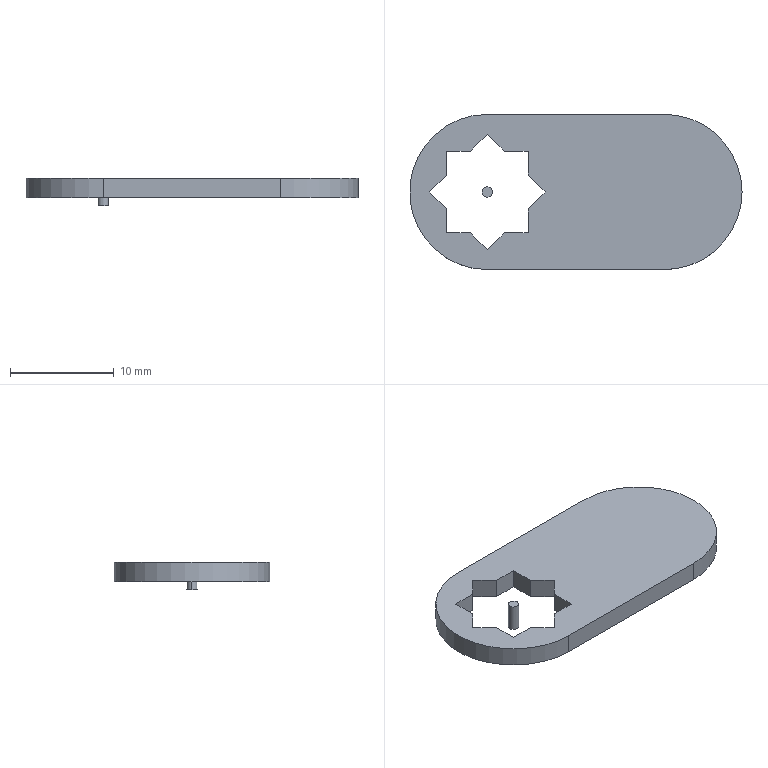Component | SolidWorks | PC-CAJ-P08-1_Lengueta Chapa Guantera Duesco B-1 | 2 solids | 27 faces | box 32 x 14.95 x 2.65 mm | volume 682 mm3 | plane 22 | cylinder 5 | commonest cylinder face diameters 14.95 x3 1 x2 | material Plain Carbon Steel
STEP:
#1=COLOUR_RGB('',0.7922,0.8196,0.9333);
#2=FILL_AREA_STYLE_COLOUR('',#1);
#3=FILL_AREA_STYLE('',(#2));
#4=SURFACE_STYLE_FILL_AREA(#3);
#5=SURFACE_SIDE_STYLE('',(#4));
#6=SURFACE_STYLE_USAGE(.BOTH.,#5);
#7=PRESENTATION_STYLE_ASSIGNMENT((#6));
#8=CARTESIAN_POINT('',(-1.142,-0.9449,8.203));
#9=VERTEX_POINT('',#8);
#10=CARTESIAN_POINT('',(-1.102,-0.9449,8.203));
#11=VERTEX_POINT('',#10);
#12=CARTESIAN_POINT('',(-1.122,-0.9449,8.203));
#13=DIRECTION('',(0.,-0.,1.));
#14=DIRECTION('',(-1.,0.,0.));
#15=AXIS2_PLACEMENT_3D('',#12,#13,#14);
#16=CIRCLE('',#15,0.01969);
#17=EDGE_CURVE('',#9,#11,#16,.T.);
#18=ORIENTED_EDGE('',*,*,#17,.T.);
#19=CARTESIAN_POINT('',(-1.102,-0.9449,8.307));
#20=VERTEX_POINT('',#19);
#21=CARTESIAN_POINT('',(-1.102,-0.9449,8.203));
#22=DIRECTION('',(0.,-0.,1.));
#23=VECTOR('',#22,39.37);
#24=LINE('',#21,#23);
#25=EDGE_CURVE('',#11,#20,#24,.T.);
#26=ORIENTED_EDGE('',*,*,#25,.T.);
#27=CARTESIAN_POINT('',(-1.142,-0.9449,8.307));
#28=VERTEX_POINT('',#27);
#29=CARTESIAN_POINT('',(-1.122,-0.9449,8.307));
#30=DIRECTION('',(-0.,0.,-1.));
#31=DIRECTION('',(-1.,0.,0.));
#32=AXIS2_PLACEMENT_3D('',#29,#30,#31);
#33=CIRCLE('',#32,0.01969);
#34=EDGE_CURVE('',#20,#28,#33,.T.);
#35=ORIENTED_EDGE('',*,*,#34,.T.);
#36=CARTESIAN_POINT('',(-1.142,-0.9449,8.203));
#37=DIRECTION('',(0.,-0.,1.));
#38=VECTOR('',#37,39.37);
#39=LINE('',#36,#38);
#40=EDGE_CURVE('',#9,#28,#39,.T.);
#41=ORIENTED_EDGE('',*,*,#40,.F.);
#42=EDGE_LOOP('',(#18,#26,#35,#41));
#43=FACE_OUTER_BOUND('',#42,.T.);
#44=CARTESIAN_POINT('',(-1.122,-0.9449,8.203));
#45=DIRECTION('',(0.,-0.,1.));
#46=DIRECTION('',(-1.,0.,0.));
#47=AXIS2_PLACEMENT_3D('',#44,#45,#46);
#48=CYLINDRICAL_SURFACE('',#47,0.01969);
#49=ADVANCED_FACE('',(#43),#48,.T.);
#50=ORIENTED_EDGE('',*,*,#25,.F.);
#51=CARTESIAN_POINT('',(-1.122,-0.9449,8.203));
#52=DIRECTION('',(0.,-0.,1.));
#53=DIRECTION('',(-1.,0.,0.));
#54=AXIS2_PLACEMENT_3D('',#51,#52,#53);
#55=CIRCLE('',#54,0.01969);
#56=EDGE_CURVE('',#11,#9,#55,.T.);
#57=ORIENTED_EDGE('',*,*,#56,.T.);
#58=ORIENTED_EDGE('',*,*,#40,.T.);
#59=CARTESIAN_POINT('',(-1.122,-0.9449,8.307));
#60=DIRECTION('',(-0.,0.,-1.));
#61=DIRECTION('',(-1.,0.,0.));
#62=AXIS2_PLACEMENT_3D('',#59,#60,#61);
#63=CIRCLE('',#62,0.01969);
#64=EDGE_CURVE('',#28,#20,#63,.T.);
#65=ORIENTED_EDGE('',*,*,#64,.T.);
#66=EDGE_LOOP('',(#50,#57,#58,#65));
#67=FACE_OUTER_BOUND('',#66,.T.);
#68=CARTESIAN_POINT('',(-1.122,-0.9449,8.203));
#69=DIRECTION('',(0.,-0.,1.));
#70=DIRECTION('',(-1.,0.,0.));
#71=AXIS2_PLACEMENT_3D('',#68,#69,#70);
#72=CYLINDRICAL_SURFACE('',#71,0.01969);
#73=ADVANCED_FACE('',(#67),#72,.T.);
#74=ORIENTED_EDGE('',*,*,#64,.F.);
#75=ORIENTED_EDGE('',*,*,#34,.F.);
#76=EDGE_LOOP('',(#74,#75));
#77=FACE_OUTER_BOUND('',#76,.T.);
#78=CARTESIAN_POINT('',(-1.102,-0.9248,8.307));
#79=DIRECTION('',(0.,-0.,1.));
#80=DIRECTION('',(-1.,0.,0.));
#81=AXIS2_PLACEMENT_3D('',#78,#79,#80);
#82=PLANE('',#81);
#83=ADVANCED_FACE('',(#77),#82,.T.);
#84=ORIENTED_EDGE('',*,*,#17,.F.);
#85=ORIENTED_EDGE('',*,*,#56,.F.);
#86=EDGE_LOOP('',(#84,#85));
#87=FACE_OUTER_BOUND('',#86,.T.);
#88=CARTESIAN_POINT('',(-1.142,-0.9248,8.203));
#89=DIRECTION('',(-0.,0.,-1.));
#90=DIRECTION('',(1.,-0.,-0.));
#91=AXIS2_PLACEMENT_3D('',#88,#89,#90);
#92=PLANE('',#91);
#93=ADVANCED_FACE('',(#87),#92,.T.);
#94=CLOSED_SHELL('',(#49,#73,#83,#93));
#95=MANIFOLD_SOLID_BREP('',#94);
#96=STYLED_ITEM('',(#7),#95);
#97=PRESENTATION_LAYER_ASSIGNMENT('','',(#96));
#98=COLOUR_RGB('',0.7922,0.8196,0.9333);
#99=FILL_AREA_STYLE_COLOUR('',#98);
#100=FILL_AREA_STYLE('',(#99));
#101=SURFACE_STYLE_FILL_AREA(#100);
#102=SURFACE_SIDE_STYLE('',(#101));
#103=SURFACE_STYLE_USAGE(.BOTH.,#102);
#104=PRESENTATION_STYLE_ASSIGNMENT((#103));
#105=CARTESIAN_POINT('',(-0.1565,-0.9449,8.307));
#106=VERTEX_POINT('',#105);
#107=CARTESIAN_POINT('',(-0.4508,-0.6506,8.307));
#108=VERTEX_POINT('',#107);
#109=CARTESIAN_POINT('',(-0.4508,-0.9449,8.307));
#110=DIRECTION('',(0.,-0.,1.));
#111=DIRECTION('',(1.,0.,0.));
#112=AXIS2_PLACEMENT_3D('',#109,#110,#111);
#113=CIRCLE('',#112,0.2943);
#114=EDGE_CURVE('',#106,#108,#113,.T.);
#115=ORIENTED_EDGE('',*,*,#114,.F.);
#116=CARTESIAN_POINT('',(-0.1565,-0.9449,8.232));
#117=VERTEX_POINT('',#116);
#118=CARTESIAN_POINT('',(-0.1565,-0.9449,8.307));
#119=DIRECTION('',(-0.,0.,-1.));
#120=VECTOR('',#119,39.37);
#121=LINE('',#118,#120);
#122=EDGE_CURVE('',#106,#117,#121,.T.);
#123=ORIENTED_EDGE('',*,*,#122,.T.);
#124=CARTESIAN_POINT('',(-0.4508,-0.6506,8.232));
#125=VERTEX_POINT('',#124);
#126=CARTESIAN_POINT('',(-0.4508,-0.9449,8.232));
#127=DIRECTION('',(-0.,0.,-1.));
#128=DIRECTION('',(1.,0.,0.));
#129=AXIS2_PLACEMENT_3D('',#126,#127,#128);
#130=CIRCLE('',#129,0.2943);
#131=EDGE_CURVE('',#125,#117,#130,.T.);
#132=ORIENTED_EDGE('',*,*,#131,.F.);
#133=CARTESIAN_POINT('',(-0.4508,-0.6506,8.27));
#134=DIRECTION('',(-0.,0.,-1.));
#135=VECTOR('',#134,39.37);
#136=LINE('',#133,#135);
#137=EDGE_CURVE('',#108,#125,#136,.T.);
#138=ORIENTED_EDGE('',*,*,#137,.F.);
#139=EDGE_LOOP('',(#115,#123,#132,#138));
#140=FACE_OUTER_BOUND('',#139,.T.);
#141=CARTESIAN_POINT('',(-0.4508,-0.9449,8.307));
#142=DIRECTION('',(-0.,0.,-1.));
#143=DIRECTION('',(1.,0.,0.));
#144=AXIS2_PLACEMENT_3D('',#141,#142,#143);
#145=CYLINDRICAL_SURFACE('',#144,0.2943);
#146=ADVANCED_FACE('',(#140),#145,.T.);
#147=CARTESIAN_POINT('',(-0.9671,-0.79,8.232));
#148=VERTEX_POINT('',#147);
#149=CARTESIAN_POINT('',(-0.9671,-0.79,8.307));
#150=VERTEX_POINT('',#149);
#151=CARTESIAN_POINT('',(-0.9671,-0.79,8.27));
#152=DIRECTION('',(0.,-0.,1.));
#153=VECTOR('',#152,39.37);
#154=LINE('',#151,#153);
#155=EDGE_CURVE('',#148,#150,#154,.T.);
#156=ORIENTED_EDGE('',*,*,#155,.T.);
#157=CARTESIAN_POINT('',(-1.058,-0.79,8.307));
#158=VERTEX_POINT('',#157);
#159=CARTESIAN_POINT('',(-1.013,-0.79,8.307));
#160=DIRECTION('',(-1.,0.,0.));
#161=VECTOR('',#160,39.37);
#162=LINE('',#159,#161);
#163=EDGE_CURVE('',#150,#158,#162,.T.);
#164=ORIENTED_EDGE('',*,*,#163,.T.);
#165=CARTESIAN_POINT('',(-1.058,-0.79,8.232));
#166=VERTEX_POINT('',#165);
#167=CARTESIAN_POINT('',(-1.058,-0.79,8.27));
#168=DIRECTION('',(-0.,0.,-1.));
#169=VECTOR('',#168,39.37);
#170=LINE('',#167,#169);
#171=EDGE_CURVE('',#158,#166,#170,.T.);
#172=ORIENTED_EDGE('',*,*,#171,.T.);
#173=CARTESIAN_POINT('',(-1.013,-0.79,8.232));
#174=DIRECTION('',(1.,-0.,-0.));
#175=VECTOR('',#174,39.37);
#176=LINE('',#173,#175);
#177=EDGE_CURVE('',#166,#148,#176,.T.);
#178=ORIENTED_EDGE('',*,*,#177,.T.);
#179=EDGE_LOOP('',(#156,#164,#172,#178));
#180=FACE_OUTER_BOUND('',#179,.T.);
#181=CARTESIAN_POINT('',(-0.9671,-0.79,8.307));
#182=DIRECTION('',(-0.,-1.,-0.));
#183=DIRECTION('',(-1.,0.,0.));
#184=AXIS2_PLACEMENT_3D('',#181,#182,#183);
#185=PLANE('',#184);
#186=ADVANCED_FACE('',(#180),#185,.T.);
#187=CARTESIAN_POINT('',(-0.9671,-0.8807,8.307));
#188=VERTEX_POINT('',#187);
#189=CARTESIAN_POINT('',(-0.903,-0.9449,8.307));
#190=VERTEX_POINT('',#189);
#191=CARTESIAN_POINT('',(-0.9671,-0.8807,8.307));
#192=DIRECTION('',(0.7071,-0.7071,-0.));
#193=VECTOR('',#192,39.37);
#194=LINE('',#191,#193);
#195=EDGE_CURVE('',#188,#190,#194,.T.);
#196=ORIENTED_EDGE('',*,*,#195,.T.);
#197=CARTESIAN_POINT('',(-0.9671,-1.009,8.307));
#198=VERTEX_POINT('',#197);
#199=CARTESIAN_POINT('',(-0.903,-0.9449,8.307));
#200=DIRECTION('',(-0.7071,-0.7071,-0.));
#201=VECTOR('',#200,39.37);
#202=LINE('',#199,#201);
#203=EDGE_CURVE('',#190,#198,#202,.T.);
#204=ORIENTED_EDGE('',*,*,#203,.T.);
#205=CARTESIAN_POINT('',(-0.9671,-1.1,8.307));
#206=VERTEX_POINT('',#205);
#207=CARTESIAN_POINT('',(-0.9671,-0.9449,8.307));
#208=DIRECTION('',(-0.,-1.,-0.));
#209=VECTOR('',#208,39.37);
#210=LINE('',#207,#209);
#211=EDGE_CURVE('',#198,#206,#210,.T.);
#212=ORIENTED_EDGE('',*,*,#211,.T.);
#213=CARTESIAN_POINT('',(-1.058,-1.1,8.307));
#214=VERTEX_POINT('',#213);
#215=CARTESIAN_POINT('',(-0.7864,-1.1,8.307));
#216=DIRECTION('',(-1.,0.,0.));
#217=VECTOR('',#216,39.37);
#218=LINE('',#215,#217);
#219=EDGE_CURVE('',#206,#214,#218,.T.);
#220=ORIENTED_EDGE('',*,*,#219,.T.);
#221=CARTESIAN_POINT('',(-1.122,-1.164,8.307));
#222=VERTEX_POINT('',#221);
#223=CARTESIAN_POINT('',(-1.058,-1.1,8.307));
#224=DIRECTION('',(-0.7071,-0.7071,-0.));
#225=VECTOR('',#224,39.37);
#226=LINE('',#223,#225);
#227=EDGE_CURVE('',#214,#222,#226,.T.);
#228=ORIENTED_EDGE('',*,*,#227,.T.);
#229=CARTESIAN_POINT('',(-1.186,-1.1,8.307));
#230=VERTEX_POINT('',#229);
#231=CARTESIAN_POINT('',(-1.122,-1.164,8.307));
#232=DIRECTION('',(-0.7071,0.7071,0.));
#233=VECTOR('',#232,39.37);
#234=LINE('',#231,#233);
#235=EDGE_CURVE('',#222,#230,#234,.T.);
#236=ORIENTED_EDGE('',*,*,#235,.T.);
#237=CARTESIAN_POINT('',(-1.277,-1.1,8.307));
#238=VERTEX_POINT('',#237);
#239=CARTESIAN_POINT('',(-0.7864,-1.1,8.307));
#240=DIRECTION('',(-1.,0.,0.));
#241=VECTOR('',#240,39.37);
#242=LINE('',#239,#241);
#243=EDGE_CURVE('',#230,#238,#242,.T.);
#244=ORIENTED_EDGE('',*,*,#243,.T.);
#245=CARTESIAN_POINT('',(-1.277,-1.009,8.307));
#246=VERTEX_POINT('',#245);
#247=CARTESIAN_POINT('',(-1.277,-0.9449,8.307));
#248=DIRECTION('',(0.,1.,0.));
#249=VECTOR('',#248,39.37);
#250=LINE('',#247,#249);
#251=EDGE_CURVE('',#238,#246,#250,.T.);
#252=ORIENTED_EDGE('',*,*,#251,.T.);
#253=CARTESIAN_POINT('',(-1.341,-0.9449,8.307));
#254=VERTEX_POINT('',#253);
#255=CARTESIAN_POINT('',(-1.277,-1.009,8.307));
#256=DIRECTION('',(-0.7071,0.7071,0.));
#257=VECTOR('',#256,39.37);
#258=LINE('',#255,#257);
#259=EDGE_CURVE('',#246,#254,#258,.T.);
#260=ORIENTED_EDGE('',*,*,#259,.T.);
#261=CARTESIAN_POINT('',(-1.277,-0.8807,8.307));
#262=VERTEX_POINT('',#261);
#263=CARTESIAN_POINT('',(-1.341,-0.9449,8.307));
#264=DIRECTION('',(0.7071,0.7071,0.));
#265=VECTOR('',#264,39.37);
#266=LINE('',#263,#265);
#267=EDGE_CURVE('',#254,#262,#266,.T.);
#268=ORIENTED_EDGE('',*,*,#267,.T.);
#269=CARTESIAN_POINT('',(-1.277,-0.79,8.307));
#270=VERTEX_POINT('',#269);
#271=CARTESIAN_POINT('',(-1.277,-0.9449,8.307));
#272=DIRECTION('',(0.,1.,0.));
#273=VECTOR('',#272,39.37);
#274=LINE('',#271,#273);
#275=EDGE_CURVE('',#262,#270,#274,.T.);
#276=ORIENTED_EDGE('',*,*,#275,.T.);
#277=CARTESIAN_POINT('',(-1.186,-0.79,8.307));
#278=VERTEX_POINT('',#277);
#279=CARTESIAN_POINT('',(-0.7864,-0.79,8.307));
#280=DIRECTION('',(1.,-0.,-0.));
#281=VECTOR('',#280,39.37);
#282=LINE('',#279,#281);
#283=EDGE_CURVE('',#270,#278,#282,.T.);
#284=ORIENTED_EDGE('',*,*,#283,.T.);
#285=CARTESIAN_POINT('',(-1.122,-0.7258,8.307));
#286=VERTEX_POINT('',#285);
#287=CARTESIAN_POINT('',(-1.186,-0.79,8.307));
#288=DIRECTION('',(0.7071,0.7071,0.));
#289=VECTOR('',#288,39.37);
#290=LINE('',#287,#289);
#291=EDGE_CURVE('',#278,#286,#290,.T.);
#292=ORIENTED_EDGE('',*,*,#291,.T.);
#293=CARTESIAN_POINT('',(-1.122,-0.7258,8.307));
#294=DIRECTION('',(0.7071,-0.7071,-0.));
#295=VECTOR('',#294,39.37);
#296=LINE('',#293,#295);
#297=EDGE_CURVE('',#286,#158,#296,.T.);
#298=ORIENTED_EDGE('',*,*,#297,.T.);
#299=ORIENTED_EDGE('',*,*,#163,.F.);
#300=CARTESIAN_POINT('',(-0.9671,-0.9449,8.307));
#301=DIRECTION('',(-0.,-1.,-0.));
#302=VECTOR('',#301,39.37);
#303=LINE('',#300,#302);
#304=EDGE_CURVE('',#150,#188,#303,.T.);
#305=ORIENTED_EDGE('',*,*,#304,.T.);
#306=EDGE_LOOP('',(#196,#204,#212,#220,#228,#236,#244,#252,#260,#268,#276,#284,#292,#298,#299,#305));
#307=FACE_BOUND('',#306,.T.);
#308=CARTESIAN_POINT('',(-1.122,-0.6506,8.307));
#309=VERTEX_POINT('',#308);
#310=CARTESIAN_POINT('',(-1.122,-1.239,8.307));
#311=VERTEX_POINT('',#310);
#312=CARTESIAN_POINT('',(-1.122,-0.9449,8.307));
#313=DIRECTION('',(0.,-0.,1.));
#314=DIRECTION('',(1.,0.,0.));
#315=AXIS2_PLACEMENT_3D('',#312,#313,#314);
#316=CIRCLE('',#315,0.2943);
#317=EDGE_CURVE('',#309,#311,#316,.T.);
#318=ORIENTED_EDGE('',*,*,#317,.T.);
#319=CARTESIAN_POINT('',(-0.4508,-1.239,8.307));
#320=VERTEX_POINT('',#319);
#321=CARTESIAN_POINT('',(-0.7864,-1.239,8.307));
#322=DIRECTION('',(1.,-0.,-0.));
#323=VECTOR('',#322,39.37);
#324=LINE('',#321,#323);
#325=EDGE_CURVE('',#311,#320,#324,.T.);
#326=ORIENTED_EDGE('',*,*,#325,.T.);
#327=CARTESIAN_POINT('',(-0.4508,-0.9449,8.307));
#328=DIRECTION('',(0.,-0.,1.));
#329=DIRECTION('',(1.,0.,0.));
#330=AXIS2_PLACEMENT_3D('',#327,#328,#329);
#331=CIRCLE('',#330,0.2943);
#332=EDGE_CURVE('',#320,#106,#331,.T.);
#333=ORIENTED_EDGE('',*,*,#332,.T.);
#334=ORIENTED_EDGE('',*,*,#114,.T.);
#335=CARTESIAN_POINT('',(-0.7864,-0.6506,8.307));
#336=DIRECTION('',(-1.,0.,0.));
#337=VECTOR('',#336,39.37);
#338=LINE('',#335,#337);
#339=EDGE_CURVE('',#108,#309,#338,.T.);
#340=ORIENTED_EDGE('',*,*,#339,.T.);
#341=EDGE_LOOP('',(#318,#326,#333,#334,#340));
#342=FACE_OUTER_BOUND('',#341,.T.);
#343=CARTESIAN_POINT('',(-0.1439,-0.6506,8.307));
#344=DIRECTION('',(0.,-0.,1.));
#345=DIRECTION('',(-1.,0.,0.));
#346=AXIS2_PLACEMENT_3D('',#343,#344,#345);
#347=PLANE('',#346);
#348=ADVANCED_FACE('',(#307,#342),#347,.T.);
#349=ORIENTED_EDGE('',*,*,#155,.F.);
#350=CARTESIAN_POINT('',(-0.9671,-0.8807,8.232));
#351=VERTEX_POINT('',#350);
#352=CARTESIAN_POINT('',(-0.9671,-0.8353,8.232));
#353=DIRECTION('',(-0.,-1.,-0.));
#354=VECTOR('',#353,39.37);
#355=LINE('',#352,#354);
#356=EDGE_CURVE('',#148,#351,#355,.T.);
#357=ORIENTED_EDGE('',*,*,#356,.T.);
#358=CARTESIAN_POINT('',(-0.9671,-0.8807,8.27));
#359=DIRECTION('',(0.,-0.,1.));
#360=VECTOR('',#359,39.37);
#361=LINE('',#358,#360);
#362=EDGE_CURVE('',#351,#188,#361,.T.);
#363=ORIENTED_EDGE('',*,*,#362,.T.);
#364=ORIENTED_EDGE('',*,*,#304,.F.);
#365=EDGE_LOOP('',(#349,#357,#363,#364));
#366=FACE_OUTER_BOUND('',#365,.T.);
#367=CARTESIAN_POINT('',(-0.9671,-0.8807,8.307));
#368=DIRECTION('',(-1.,0.,0.));
#369=DIRECTION('',(0.,1.,0.));
#370=AXIS2_PLACEMENT_3D('',#367,#368,#369);
#371=PLANE('',#370);
#372=ADVANCED_FACE('',(#366),#371,.T.);
#373=CARTESIAN_POINT('',(-1.122,-1.164,8.232));
#374=VERTEX_POINT('',#373);
#375=CARTESIAN_POINT('',(-1.058,-1.1,8.232));
#376=VERTEX_POINT('',#375);
#377=CARTESIAN_POINT('',(-1.122,-1.164,8.232));
#378=DIRECTION('',(0.7071,0.7071,0.));
#379=VECTOR('',#378,39.37);
#380=LINE('',#377,#379);
#381=EDGE_CURVE('',#374,#376,#380,.T.);
#382=ORIENTED_EDGE('',*,*,#381,.T.);
#383=CARTESIAN_POINT('',(-0.9671,-1.1,8.232));
#384=VERTEX_POINT('',#383);
#385=CARTESIAN_POINT('',(-0.7864,-1.1,8.232));
#386=DIRECTION('',(1.,-0.,-0.));
#387=VECTOR('',#386,39.37);
#388=LINE('',#385,#387);
#389=EDGE_CURVE('',#376,#384,#388,.T.);
#390=ORIENTED_EDGE('',*,*,#389,.T.);
#391=CARTESIAN_POINT('',(-0.9671,-1.009,8.232));
#392=VERTEX_POINT('',#391);
#393=CARTESIAN_POINT('',(-0.9671,-0.9449,8.232));
#394=DIRECTION('',(0.,1.,0.));
#395=VECTOR('',#394,39.37);
#396=LINE('',#393,#395);
#397=EDGE_CURVE('',#384,#392,#396,.T.);
#398=ORIENTED_EDGE('',*,*,#397,.T.);
#399=CARTESIAN_POINT('',(-0.903,-0.9449,8.232));
#400=VERTEX_POINT('',#399);
#401=CARTESIAN_POINT('',(-0.9671,-1.009,8.232));
#402=DIRECTION('',(0.7071,0.7071,0.));
#403=VECTOR('',#402,39.37);
#404=LINE('',#401,#403);
#405=EDGE_CURVE('',#392,#400,#404,.T.);
#406=ORIENTED_EDGE('',*,*,#405,.T.);
#407=CARTESIAN_POINT('',(-0.903,-0.9449,8.232));
#408=DIRECTION('',(-0.7071,0.7071,0.));
#409=VECTOR('',#408,39.37);
#410=LINE('',#407,#409);
#411=EDGE_CURVE('',#400,#351,#410,.T.);
#412=ORIENTED_EDGE('',*,*,#411,.T.);
#413=ORIENTED_EDGE('',*,*,#356,.F.);
#414=ORIENTED_EDGE('',*,*,#177,.F.);
#415=CARTESIAN_POINT('',(-1.122,-0.7258,8.232));
#416=VERTEX_POINT('',#415);
#417=CARTESIAN_POINT('',(-1.058,-0.79,8.232));
#418=DIRECTION('',(-0.7071,0.7071,0.));
#419=VECTOR('',#418,39.37);
#420=LINE('',#417,#419);
#421=EDGE_CURVE('',#166,#416,#420,.T.);
#422=ORIENTED_EDGE('',*,*,#421,.T.);
#423=CARTESIAN_POINT('',(-1.186,-0.79,8.232));
#424=VERTEX_POINT('',#423);
#425=CARTESIAN_POINT('',(-1.122,-0.7258,8.232));
#426=DIRECTION('',(-0.7071,-0.7071,-0.));
#427=VECTOR('',#426,39.37);
#428=LINE('',#425,#427);
#429=EDGE_CURVE('',#416,#424,#428,.T.);
#430=ORIENTED_EDGE('',*,*,#429,.T.);
#431=CARTESIAN_POINT('',(-1.277,-0.79,8.232));
#432=VERTEX_POINT('',#431);
#433=CARTESIAN_POINT('',(-0.7864,-0.79,8.232));
#434=DIRECTION('',(-1.,0.,0.));
#435=VECTOR('',#434,39.37);
#436=LINE('',#433,#435);
#437=EDGE_CURVE('',#424,#432,#436,.T.);
#438=ORIENTED_EDGE('',*,*,#437,.T.);
#439=CARTESIAN_POINT('',(-1.277,-0.8807,8.232));
#440=VERTEX_POINT('',#439);
#441=CARTESIAN_POINT('',(-1.277,-0.9449,8.232));
#442=DIRECTION('',(-0.,-1.,-0.));
#443=VECTOR('',#442,39.37);
#444=LINE('',#441,#443);
#445=EDGE_CURVE('',#432,#440,#444,.T.);
#446=ORIENTED_EDGE('',*,*,#445,.T.);
#447=CARTESIAN_POINT('',(-1.341,-0.9449,8.232));
#448=VERTEX_POINT('',#447);
#449=CARTESIAN_POINT('',(-1.277,-0.8807,8.232));
#450=DIRECTION('',(-0.7071,-0.7071,-0.));
#451=VECTOR('',#450,39.37);
#452=LINE('',#449,#451);
#453=EDGE_CURVE('',#440,#448,#452,.T.);
#454=ORIENTED_EDGE('',*,*,#453,.T.);
#455=CARTESIAN_POINT('',(-1.277,-1.009,8.232));
#456=VERTEX_POINT('',#455);
#457=CARTESIAN_POINT('',(-1.341,-0.9449,8.232));
#458=DIRECTION('',(0.7071,-0.7071,-0.));
#459=VECTOR('',#458,39.37);
#460=LINE('',#457,#459);
#461=EDGE_CURVE('',#448,#456,#460,.T.);
#462=ORIENTED_EDGE('',*,*,#461,.T.);
#463=CARTESIAN_POINT('',(-1.277,-1.1,8.232));
#464=VERTEX_POINT('',#463);
#465=CARTESIAN_POINT('',(-1.277,-0.9449,8.232));
#466=DIRECTION('',(-0.,-1.,-0.));
#467=VECTOR('',#466,39.37);
#468=LINE('',#465,#467);
#469=EDGE_CURVE('',#456,#464,#468,.T.);
#470=ORIENTED_EDGE('',*,*,#469,.T.);
#471=CARTESIAN_POINT('',(-1.186,-1.1,8.232));
#472=VERTEX_POINT('',#471);
#473=CARTESIAN_POINT('',(-0.7864,-1.1,8.232));
#474=DIRECTION('',(1.,-0.,-0.));
#475=VECTOR('',#474,39.37);
#476=LINE('',#473,#475);
#477=EDGE_CURVE('',#464,#472,#476,.T.);
#478=ORIENTED_EDGE('',*,*,#477,.T.);
#479=CARTESIAN_POINT('',(-1.186,-1.1,8.232));
#480=DIRECTION('',(0.7071,-0.7071,-0.));
#481=VECTOR('',#480,39.37);
#482=LINE('',#479,#481);
#483=EDGE_CURVE('',#472,#374,#482,.T.);
#484=ORIENTED_EDGE('',*,*,#483,.T.);
#485=EDGE_LOOP('',(#382,#390,#398,#406,#412,#413,#414,#422,#430,#438,#446,#454,#462,#470,#478,#484));
#486=FACE_BOUND('',#485,.T.);
#487=CARTESIAN_POINT('',(-1.122,-1.239,8.232));
#488=VERTEX_POINT('',#487);
#489=CARTESIAN_POINT('',(-1.122,-0.6506,8.232));
#490=VERTEX_POINT('',#489);
#491=CARTESIAN_POINT('',(-1.122,-0.9449,8.232));
#492=DIRECTION('',(-0.,0.,-1.));
#493=DIRECTION('',(1.,0.,0.));
#494=AXIS2_PLACEMENT_3D('',#491,#492,#493);
#495=CIRCLE('',#494,0.2943);
#496=EDGE_CURVE('',#488,#490,#495,.T.);
#497=ORIENTED_EDGE('',*,*,#496,.T.);
#498=CARTESIAN_POINT('',(-0.7864,-0.6506,8.232));
#499=DIRECTION('',(1.,-0.,-0.));
#500=VECTOR('',#499,39.37);
#501=LINE('',#498,#500);
#502=EDGE_CURVE('',#490,#125,#501,.T.);
#503=ORIENTED_EDGE('',*,*,#502,.T.);
#504=ORIENTED_EDGE('',*,*,#131,.T.);
#505=CARTESIAN_POINT('',(-0.4508,-1.239,8.232));
#506=VERTEX_POINT('',#505);
#507=CARTESIAN_POINT('',(-0.4508,-0.9449,8.232));
#508=DIRECTION('',(-0.,0.,-1.));
#509=DIRECTION('',(1.,0.,0.));
#510=AXIS2_PLACEMENT_3D('',#507,#508,#509);
#511=CIRCLE('',#510,0.2943);
#512=EDGE_CURVE('',#117,#506,#511,.T.);
#513=ORIENTED_EDGE('',*,*,#512,.T.);
#514=CARTESIAN_POINT('',(-0.7864,-1.239,8.232));
#515=DIRECTION('',(-1.,0.,0.));
#516=VECTOR('',#515,39.37);
#517=LINE('',#514,#516);
#518=EDGE_CURVE('',#506,#488,#517,.T.);
#519=ORIENTED_EDGE('',*,*,#518,.T.);
#520=EDGE_LOOP('',(#497,#503,#504,#513,#519));
#521=FACE_OUTER_BOUND('',#520,.T.);
#522=CARTESIAN_POINT('',(-1.429,-0.6506,8.232));
#523=DIRECTION('',(-0.,0.,-1.));
#524=DIRECTION('',(1.,-0.,-0.));
#525=AXIS2_PLACEMENT_3D('',#522,#523,#524);
#526=PLANE('',#525);
#527=ADVANCED_FACE('',(#486,#521),#526,.T.);
#528=CARTESIAN_POINT('',(-1.122,-0.7258,8.27));
#529=DIRECTION('',(-0.,0.,-1.));
#530=VECTOR('',#529,39.37);
#531=LINE('',#528,#530);
#532=EDGE_CURVE('',#286,#416,#531,.T.);
#533=ORIENTED_EDGE('',*,*,#532,.T.);
#534=ORIENTED_EDGE('',*,*,#421,.F.);
#535=ORIENTED_EDGE('',*,*,#171,.F.);
#536=ORIENTED_EDGE('',*,*,#297,.F.);
#537=EDGE_LOOP('',(#533,#534,#535,#536));
#538=FACE_OUTER_BOUND('',#537,.T.);
#539=CARTESIAN_POINT('',(-1.058,-0.79,8.307));
#540=DIRECTION('',(-0.7071,-0.7071,-0.));
#541=DIRECTION('',(-0.7071,0.7071,0.));
#542=AXIS2_PLACEMENT_3D('',#539,#540,#541);
#543=PLANE('',#542);
#544=ADVANCED_FACE('',(#538),#543,.T.);
#545=CARTESIAN_POINT('',(-0.903,-0.9449,8.27));
#546=DIRECTION('',(-0.,0.,-1.));
#547=VECTOR('',#546,39.37);
#548=LINE('',#545,#547);
#549=EDGE_CURVE('',#190,#400,#548,.T.);
#550=ORIENTED_EDGE('',*,*,#549,.T.);
#551=ORIENTED_EDGE('',*,*,#405,.F.);
#552=CARTESIAN_POINT('',(-0.9671,-1.009,8.27));
#553=DIRECTION('',(0.,-0.,1.));
#554=VECTOR('',#553,39.37);
#555=LINE('',#552,#554);
#556=EDGE_CURVE('',#392,#198,#555,.T.);
#557=ORIENTED_EDGE('',*,*,#556,.T.);
#558=ORIENTED_EDGE('',*,*,#203,.F.);
#559=EDGE_LOOP('',(#550,#551,#557,#558));
#560=FACE_OUTER_BOUND('',#559,.T.);
#561=CARTESIAN_POINT('',(-0.9671,-1.009,8.307));
#562=DIRECTION('',(-0.7071,0.7071,0.));
#563=DIRECTION('',(0.7071,0.7071,0.));
#564=AXIS2_PLACEMENT_3D('',#561,#562,#563);
#565=PLANE('',#564);
#566=ADVANCED_FACE('',(#560),#565,.T.);
#567=ORIENTED_EDGE('',*,*,#549,.F.);
#568=ORIENTED_EDGE('',*,*,#195,.F.);
#569=ORIENTED_EDGE('',*,*,#362,.F.);
#570=ORIENTED_EDGE('',*,*,#411,.F.);
#571=EDGE_LOOP('',(#567,#568,#569,#570));
#572=FACE_OUTER_BOUND('',#571,.T.);
#573=CARTESIAN_POINT('',(-0.903,-0.9449,8.307));
#574=DIRECTION('',(-0.7071,-0.7071,-0.));
#575=DIRECTION('',(-0.7071,0.7071,0.));
#576=AXIS2_PLACEMENT_3D('',#573,#574,#575);
#577=PLANE('',#576);
#578=ADVANCED_FACE('',(#572),#577,.T.);
#579=ORIENTED_EDGE('',*,*,#532,.F.);
#580=ORIENTED_EDGE('',*,*,#291,.F.);
#581=CARTESIAN_POINT('',(-1.186,-0.79,8.27));
#582=DIRECTION('',(-0.,0.,-1.));
#583=VECTOR('',#582,39.37);
#584=LINE('',#581,#583);
#585=EDGE_CURVE('',#278,#424,#584,.T.);
#586=ORIENTED_EDGE('',*,*,#585,.T.);
#587=ORIENTED_EDGE('',*,*,#429,.F.);
#588=EDGE_LOOP('',(#579,#580,#586,#587));
#589=FACE_OUTER_BOUND('',#588,.T.);
#590=CARTESIAN_POINT('',(-1.122,-0.7258,8.307));
#591=DIRECTION('',(0.7071,-0.7071,-0.));
#592=DIRECTION('',(-0.7071,-0.7071,-0.));
#593=AXIS2_PLACEMENT_3D('',#590,#591,#592);
#594=PLANE('',#593);
#595=ADVANCED_FACE('',(#589),#594,.T.);
#596=CARTESIAN_POINT('',(-1.277,-0.79,8.27));
#597=DIRECTION('',(-0.,0.,-1.));
#598=VECTOR('',#597,39.37);
#599=LINE('',#596,#598);
#600=EDGE_CURVE('',#270,#432,#599,.T.);
#601=ORIENTED_EDGE('',*,*,#600,.T.);
#602=ORIENTED_EDGE('',*,*,#437,.F.);
#603=ORIENTED_EDGE('',*,*,#585,.F.);
#604=ORIENTED_EDGE('',*,*,#283,.F.);
#605=EDGE_LOOP('',(#601,#602,#603,#604));
#606=FACE_OUTER_BOUND('',#605,.T.);
#607=CARTESIAN_POINT('',(-1.186,-0.79,8.307));
#608=DIRECTION('',(-0.,-1.,-0.));
#609=DIRECTION('',(-1.,0.,0.));
#610=AXIS2_PLACEMENT_3D('',#607,#608,#609);
#611=PLANE('',#610);
#612=ADVANCED_FACE('',(#606),#611,.T.);
#613=ORIENTED_EDGE('',*,*,#600,.F.);
#614=ORIENTED_EDGE('',*,*,#275,.F.);
#615=CARTESIAN_POINT('',(-1.277,-0.8807,8.27));
#616=DIRECTION('',(-0.,0.,-1.));
#617=VECTOR('',#616,39.37);
#618=LINE('',#615,#617);
#619=EDGE_CURVE('',#262,#440,#618,.T.);
#620=ORIENTED_EDGE('',*,*,#619,.T.);
#621=ORIENTED_EDGE('',*,*,#445,.F.);
#622=EDGE_LOOP('',(#613,#614,#620,#621));
#623=FACE_OUTER_BOUND('',#622,.T.);
#624=CARTESIAN_POINT('',(-1.277,-0.79,8.307));
#625=DIRECTION('',(1.,-0.,-0.));
#626=DIRECTION('',(-0.,-1.,-0.));
#627=AXIS2_PLACEMENT_3D('',#624,#625,#626);
#628=PLANE('',#627);
#629=ADVANCED_FACE('',(#623),#628,.T.);
#630=CARTESIAN_POINT('',(-1.341,-0.9449,8.27));
#631=DIRECTION('',(-0.,0.,-1.));
#632=VECTOR('',#631,39.37);
#633=LINE('',#630,#632);
#634=EDGE_CURVE('',#254,#448,#633,.T.);
#635=ORIENTED_EDGE('',*,*,#634,.T.);
#636=ORIENTED_EDGE('',*,*,#453,.F.);
#637=ORIENTED_EDGE('',*,*,#619,.F.);
#638=ORIENTED_EDGE('',*,*,#267,.F.);
#639=EDGE_LOOP('',(#635,#636,#637,#638));
#640=FACE_OUTER_BOUND('',#639,.T.);
#641=CARTESIAN_POINT('',(-1.277,-0.8807,8.307));
#642=DIRECTION('',(0.7071,-0.7071,-0.));
#643=DIRECTION('',(-0.7071,-0.7071,-0.));
#644=AXIS2_PLACEMENT_3D('',#641,#642,#643);
#645=PLANE('',#644);
#646=ADVANCED_FACE('',(#640),#645,.T.);
#647=ORIENTED_EDGE('',*,*,#634,.F.);
#648=ORIENTED_EDGE('',*,*,#259,.F.);
#649=CARTESIAN_POINT('',(-1.277,-1.009,8.27));
#650=DIRECTION('',(-0.,0.,-1.));
#651=VECTOR('',#650,39.37);
#652=LINE('',#649,#651);
#653=EDGE_CURVE('',#246,#456,#652,.T.);
#654=ORIENTED_EDGE('',*,*,#653,.T.);
#655=ORIENTED_EDGE('',*,*,#461,.F.);
#656=EDGE_LOOP('',(#647,#648,#654,#655));
#657=FACE_OUTER_BOUND('',#656,.T.);
#658=CARTESIAN_POINT('',(-1.341,-0.9449,8.307));
#659=DIRECTION('',(0.7071,0.7071,0.));
#660=DIRECTION('',(0.7071,-0.7071,-0.));
#661=AXIS2_PLACEMENT_3D('',#658,#659,#660);
#662=PLANE('',#661);
#663=ADVANCED_FACE('',(#657),#662,.T.);
#664=CARTESIAN_POINT('',(-1.277,-1.1,8.27));
#665=DIRECTION('',(-0.,0.,-1.));
#666=VECTOR('',#665,39.37);
#667=LINE('',#664,#666);
#668=EDGE_CURVE('',#238,#464,#667,.T.);
#669=ORIENTED_EDGE('',*,*,#668,.T.);
#670=ORIENTED_EDGE('',*,*,#469,.F.);
#671=ORIENTED_EDGE('',*,*,#653,.F.);
#672=ORIENTED_EDGE('',*,*,#251,.F.);
#673=EDGE_LOOP('',(#669,#670,#671,#672));
#674=FACE_OUTER_BOUND('',#673,.T.);
#675=CARTESIAN_POINT('',(-1.277,-1.009,8.307));
#676=DIRECTION('',(1.,-0.,-0.));
#677=DIRECTION('',(-0.,-1.,-0.));
#678=AXIS2_PLACEMENT_3D('',#675,#676,#677);
#679=PLANE('',#678);
#680=ADVANCED_FACE('',(#674),#679,.T.);
#681=ORIENTED_EDGE('',*,*,#668,.F.);
#682=ORIENTED_EDGE('',*,*,#243,.F.);
#683=CARTESIAN_POINT('',(-1.186,-1.1,8.27));
#684=DIRECTION('',(-0.,0.,-1.));
#685=VECTOR('',#684,39.37);
#686=LINE('',#683,#685);
#687=EDGE_CURVE('',#230,#472,#686,.T.);
#688=ORIENTED_EDGE('',*,*,#687,.T.);
#689=ORIENTED_EDGE('',*,*,#477,.F.);
#690=EDGE_LOOP('',(#681,#682,#688,#689));
#691=FACE_OUTER_BOUND('',#690,.T.);
#692=CARTESIAN_POINT('',(-1.277,-1.1,8.307));
#693=DIRECTION('',(0.,1.,0.));
#694=DIRECTION('',(1.,-0.,-0.));
#695=AXIS2_PLACEMENT_3D('',#692,#693,#694);
#696=PLANE('',#695);
#697=ADVANCED_FACE('',(#691),#696,.T.);
#698=CARTESIAN_POINT('',(-1.122,-1.164,8.27));
#699=DIRECTION('',(-0.,0.,-1.));
#700=VECTOR('',#699,39.37);
#701=LINE('',#698,#700);
#702=EDGE_CURVE('',#222,#374,#701,.T.);
#703=ORIENTED_EDGE('',*,*,#702,.T.);
#704=ORIENTED_EDGE('',*,*,#483,.F.);
#705=ORIENTED_EDGE('',*,*,#687,.F.);
#706=ORIENTED_EDGE('',*,*,#235,.F.);
#707=EDGE_LOOP('',(#703,#704,#705,#706));
#708=FACE_OUTER_BOUND('',#707,.T.);
#709=CARTESIAN_POINT('',(-1.186,-1.1,8.307));
#710=DIRECTION('',(0.7071,0.7071,0.));
#711=DIRECTION('',(0.7071,-0.7071,-0.));
#712=AXIS2_PLACEMENT_3D('',#709,#710,#711);
#713=PLANE('',#712);
#714=ADVANCED_FACE('',(#708),#713,.T.);
#715=ORIENTED_EDGE('',*,*,#702,.F.);
#716=ORIENTED_EDGE('',*,*,#227,.F.);
#717=CARTESIAN_POINT('',(-1.058,-1.1,8.27));
#718=DIRECTION('',(-0.,0.,-1.));
#719=VECTOR('',#718,39.37);
#720=LINE('',#717,#719);
#721=EDGE_CURVE('',#214,#376,#720,.T.);
#722=ORIENTED_EDGE('',*,*,#721,.T.);
#723=ORIENTED_EDGE('',*,*,#381,.F.);
#724=EDGE_LOOP('',(#715,#716,#722,#723));
#725=FACE_OUTER_BOUND('',#724,.T.);
#726=CARTESIAN_POINT('',(-1.122,-1.164,8.307));
#727=DIRECTION('',(-0.7071,0.7071,0.));
#728=DIRECTION('',(0.7071,0.7071,0.));
#729=AXIS2_PLACEMENT_3D('',#726,#727,#728);
#730=PLANE('',#729);
#731=ADVANCED_FACE('',(#725),#730,.T.);
#732=CARTESIAN_POINT('',(-0.9671,-1.1,8.27));
#733=DIRECTION('',(-0.,0.,-1.));
#734=VECTOR('',#733,39.37);
#735=LINE('',#732,#734);
#736=EDGE_CURVE('',#206,#384,#735,.T.);
#737=ORIENTED_EDGE('',*,*,#736,.T.);
#738=ORIENTED_EDGE('',*,*,#389,.F.);
#739=ORIENTED_EDGE('',*,*,#721,.F.);
#740=ORIENTED_EDGE('',*,*,#219,.F.);
#741=EDGE_LOOP('',(#737,#738,#739,#740));
#742=FACE_OUTER_BOUND('',#741,.T.);
#743=CARTESIAN_POINT('',(-1.058,-1.1,8.307));
#744=DIRECTION('',(0.,1.,0.));
#745=DIRECTION('',(1.,-0.,-0.));
#746=AXIS2_PLACEMENT_3D('',#743,#744,#745);
#747=PLANE('',#746);
#748=ADVANCED_FACE('',(#742),#747,.T.);
#749=ORIENTED_EDGE('',*,*,#736,.F.);
#750=ORIENTED_EDGE('',*,*,#211,.F.);
#751=ORIENTED_EDGE('',*,*,#556,.F.);
#752=ORIENTED_EDGE('',*,*,#397,.F.);
#753=EDGE_LOOP('',(#749,#750,#751,#752));
#754=FACE_OUTER_BOUND('',#753,.T.);
#755=CARTESIAN_POINT('',(-0.9671,-1.1,8.307));
#756=DIRECTION('',(-1.,0.,0.));
#757=DIRECTION('',(0.,1.,0.));
#758=AXIS2_PLACEMENT_3D('',#755,#756,#757);
#759=PLANE('',#758);
#760=ADVANCED_FACE('',(#754),#759,.T.);
#761=ORIENTED_EDGE('',*,*,#518,.F.);
#762=CARTESIAN_POINT('',(-0.4508,-1.239,8.27));
#763=DIRECTION('',(0.,-0.,1.));
#764=VECTOR('',#763,39.37);
#765=LINE('',#762,#764);
#766=EDGE_CURVE('',#506,#320,#765,.T.);
#767=ORIENTED_EDGE('',*,*,#766,.T.);
#768=ORIENTED_EDGE('',*,*,#325,.F.);
#769=CARTESIAN_POINT('',(-1.122,-1.239,8.27));
#770=DIRECTION('',(-0.,0.,-1.));
#771=VECTOR('',#770,39.37);
#772=LINE('',#769,#771);
#773=EDGE_CURVE('',#311,#488,#772,.T.);
#774=ORIENTED_EDGE('',*,*,#773,.T.);
#775=EDGE_LOOP('',(#761,#767,#768,#774));
#776=FACE_OUTER_BOUND('',#775,.T.);
#777=CARTESIAN_POINT('',(-0.4508,-1.239,8.232));
#778=DIRECTION('',(-0.,-1.,-0.));
#779=DIRECTION('',(0.,-0.,1.));
#780=AXIS2_PLACEMENT_3D('',#777,#778,#779);
#781=PLANE('',#780);
#782=ADVANCED_FACE('',(#776),#781,.T.);
#783=ORIENTED_EDGE('',*,*,#773,.F.);
#784=ORIENTED_EDGE('',*,*,#317,.F.);
#785=CARTESIAN_POINT('',(-1.122,-0.6506,8.27));
#786=DIRECTION('',(-0.,0.,-1.));
#787=VECTOR('',#786,39.37);
#788=LINE('',#785,#787);
#789=EDGE_CURVE('',#309,#490,#788,.T.);
#790=ORIENTED_EDGE('',*,*,#789,.T.);
#791=ORIENTED_EDGE('',*,*,#496,.F.);
#792=EDGE_LOOP('',(#783,#784,#790,#791));
#793=FACE_OUTER_BOUND('',#792,.T.);
#794=CARTESIAN_POINT('',(-1.122,-0.9449,8.307));
#795=DIRECTION('',(-0.,0.,-1.));
#796=DIRECTION('',(1.,0.,0.));
#797=AXIS2_PLACEMENT_3D('',#794,#795,#796);
#798=CYLINDRICAL_SURFACE('',#797,0.2943);
#799=ADVANCED_FACE('',(#793),#798,.T.);
#800=ORIENTED_EDGE('',*,*,#502,.F.);
#801=ORIENTED_EDGE('',*,*,#789,.F.);
#802=ORIENTED_EDGE('',*,*,#339,.F.);
#803=ORIENTED_EDGE('',*,*,#137,.T.);
#804=EDGE_LOOP('',(#800,#801,#802,#803));
#805=FACE_OUTER_BOUND('',#804,.T.);
#806=CARTESIAN_POINT('',(-0.4508,-0.6506,8.307));
#807=DIRECTION('',(0.,1.,0.));
#808=DIRECTION('',(-0.,0.,-1.));
#809=AXIS2_PLACEMENT_3D('',#806,#807,#808);
#810=PLANE('',#809);
#811=ADVANCED_FACE('',(#805),#810,.T.);
#812=ORIENTED_EDGE('',*,*,#122,.F.);
#813=ORIENTED_EDGE('',*,*,#332,.F.);
#814=ORIENTED_EDGE('',*,*,#766,.F.);
#815=ORIENTED_EDGE('',*,*,#512,.F.);
#816=EDGE_LOOP('',(#812,#813,#814,#815));
#817=FACE_OUTER_BOUND('',#816,.T.);
#818=CARTESIAN_POINT('',(-0.4508,-0.9449,8.307));
#819=DIRECTION('',(-0.,0.,-1.));
#820=DIRECTION('',(1.,0.,0.));
#821=AXIS2_PLACEMENT_3D('',#818,#819,#820);
#822=CYLINDRICAL_SURFACE('',#821,0.2943);
#823=ADVANCED_FACE('',(#817),#822,.T.);
#824=CLOSED_SHELL('',(#146,#186,#348,#372,#527,#544,#566,#578,#595,#612,#629,#646,#663,#680,#697,#714,#731,#748,#760,#782,#799,#811,#823));
#825=MANIFOLD_SOLID_BREP('',#824);
#826=STYLED_ITEM('',(#104),#825);
#827=PRESENTATION_LAYER_ASSIGNMENT('','',(#826));
#828=(LENGTH_UNIT()NAMED_UNIT(*)SI_UNIT($,.METRE.));
#829=LENGTH_MEASURE_WITH_UNIT(LENGTH_MEASURE(0.0254),#828);
#830=DIMENSIONAL_EXPONENTS(1.,0.,0.,0.,0.,0.,0.);
#831=(CONVERSION_BASED_UNIT('',#829)LENGTH_UNIT()NAMED_UNIT(#830));
#832=UNCERTAINTY_MEASURE_WITH_UNIT(LENGTH_MEASURE(0.00001),#831,'','');
#833=(NAMED_UNIT(*)PLANE_ANGLE_UNIT()SI_UNIT($,.RADIAN.));
#834=(NAMED_UNIT(*)SI_UNIT($,.STERADIAN.)SOLID_ANGLE_UNIT());
#835=(GEOMETRIC_REPRESENTATION_CONTEXT(3)GLOBAL_UNCERTAINTY_ASSIGNED_CONTEXT((#832))GLOBAL_UNIT_ASSIGNED_CONTEXT((#831,#833,#834))REPRESENTATION_CONTEXT('',''));
#836=MECHANICAL_DESIGN_GEOMETRIC_PRESENTATION_REPRESENTATION('',(#96),#835);
#837=(LENGTH_UNIT()NAMED_UNIT(*)SI_UNIT($,.METRE.));
#838=LENGTH_MEASURE_WITH_UNIT(LENGTH_MEASURE(0.0254),#837);
#839=DIMENSIONAL_EXPONENTS(1.,0.,0.,0.,0.,0.,0.);
#840=(CONVERSION_BASED_UNIT('',#838)LENGTH_UNIT()NAMED_UNIT(#839));
#841=UNCERTAINTY_MEASURE_WITH_UNIT(LENGTH_MEASURE(0.00001),#840,'','');
#842=(NAMED_UNIT(*)PLANE_ANGLE_UNIT()SI_UNIT($,.RADIAN.));
#843=(NAMED_UNIT(*)SI_UNIT($,.STERADIAN.)SOLID_ANGLE_UNIT());
#844=(GEOMETRIC_REPRESENTATION_CONTEXT(3)GLOBAL_UNCERTAINTY_ASSIGNED_CONTEXT((#841))GLOBAL_UNIT_ASSIGNED_CONTEXT((#840,#842,#843))REPRESENTATION_CONTEXT('',''));
#845=MECHANICAL_DESIGN_GEOMETRIC_PRESENTATION_REPRESENTATION('',(#826),#844);
#846=CARTESIAN_POINT('',(0.,0.,0.));
#847=DIRECTION('',(0.,0.,1.));
#848=DIRECTION('',(1.,0.,0.));
#849=AXIS2_PLACEMENT_3D('',#846,#847,#848);
#850=(LENGTH_UNIT()NAMED_UNIT(*)SI_UNIT($,.METRE.));
#851=LENGTH_MEASURE_WITH_UNIT(LENGTH_MEASURE(0.0254),#850);
#852=DIMENSIONAL_EXPONENTS(1.,0.,0.,0.,0.,0.,0.);
#853=(CONVERSION_BASED_UNIT('',#851)LENGTH_UNIT()NAMED_UNIT(#852));
#854=UNCERTAINTY_MEASURE_WITH_UNIT(LENGTH_MEASURE(0.00001),#853,'','');
#855=(NAMED_UNIT(*)PLANE_ANGLE_UNIT()SI_UNIT($,.RADIAN.));
#856=(NAMED_UNIT(*)SI_UNIT($,.STERADIAN.)SOLID_ANGLE_UNIT());
#857=(GEOMETRIC_REPRESENTATION_CONTEXT(3)GLOBAL_UNCERTAINTY_ASSIGNED_CONTEXT((#854))GLOBAL_UNIT_ASSIGNED_CONTEXT((#853,#855,#856))REPRESENTATION_CONTEXT('',''));
#858=ADVANCED_BREP_SHAPE_REPRESENTATION('',(#825,#95,#849),#857);